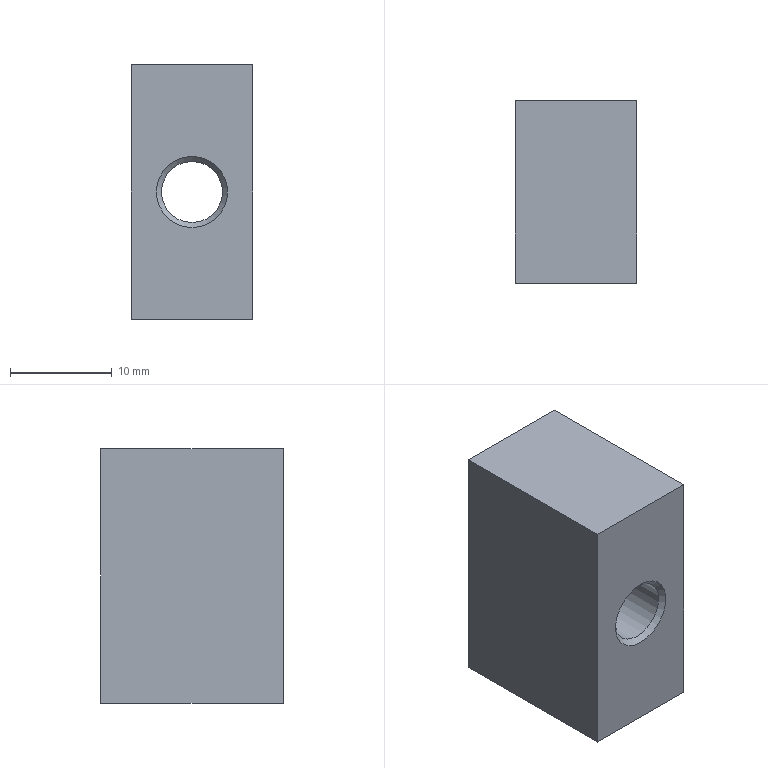Component | NX | SMALL_SLIDER | 1 solid | 9 faces | box 12 x 18 x 25 mm | volume 4886 mm3 | plane 6 | cone 2 | cylinder 1 | commonest cylinder face diameters 6 x1
STEP:
#1=CARTESIAN_POINT('',(0.,0.,0.));
#2=DIRECTION('',(0.,0.,1.));
#3=DIRECTION('',(1.,0.,0.));
#4=AXIS2_PLACEMENT_3D('',#1,#2,#3);
#5=CARTESIAN_POINT('',(-0.,-32.,1.));
#6=VERTEX_POINT('',#5);
#7=CARTESIAN_POINT('',(-0.,-32.,4.5));
#8=DIRECTION('',(0.,1.,0.));
#9=DIRECTION('',(0.,0.,-1.));
#10=AXIS2_PLACEMENT_3D('',#7,#8,#9);
#11=CIRCLE('',#10,3.5);
#12=CARTESIAN_POINT('',(6.,-32.,-8.));
#13=DIRECTION('',(0.,-1.,0.));
#14=DIRECTION('',(0.,0.,-1.));
#15=AXIS2_PLACEMENT_3D('',#12,#13,#14);
#16=PLANE('',#15);
#17=CARTESIAN_POINT('',(-9.,-6.));
#18=CARTESIAN_POINT('',(-9.,-12.062));
#19=CARTESIAN_POINT('',(-14.25,-9.031));
#20=CARTESIAN_POINT('',(-19.5,-6.));
#21=CARTESIAN_POINT('',(-14.25,-2.969));
#22=CARTESIAN_POINT('',(-9.,0.06218));
#23=CARTESIAN_POINT('',(-9.,-6.));
#24=(BOUNDED_CURVE()B_SPLINE_CURVE(2,(#17,#18,#19,#20,#21,#22,#23),.UNSPECIFIED.,.T.,.F.)B_SPLINE_CURVE_WITH_KNOTS((1,2,2,2,2,1),(-2.094,0.,2.094,4.189,6.283,8.378),.UNSPECIFIED.)CURVE()GEOMETRIC_REPRESENTATION_ITEM()RATIONAL_B_SPLINE_CURVE((1.,0.5,1.,0.5,1.,0.5,1.))REPRESENTATION_ITEM(''));
#25=(GEOMETRIC_REPRESENTATION_CONTEXT(2)PARAMETRIC_REPRESENTATION_CONTEXT()REPRESENTATION_CONTEXT('',''));
#26=DEFINITIONAL_REPRESENTATION('',(#24),#25);
#27=PCURVE('',#16,#26);
#28=CARTESIAN_POINT('',(-0.,-32.,4.5));
#29=DIRECTION('',(0.,-1.,0.));
#30=DIRECTION('',(0.,0.,-1.));
#31=AXIS2_PLACEMENT_3D('',#28,#29,#30);
#32=CONICAL_SURFACE('',#31,3.5,0.7854);
#33=CARTESIAN_POINT('',(6.283,0.));
#34=DIRECTION('',(-1.,0.));
#35=VECTOR('',#34,1.);
#36=LINE('',#33,#35);
#37=(GEOMETRIC_REPRESENTATION_CONTEXT(2)PARAMETRIC_REPRESENTATION_CONTEXT()REPRESENTATION_CONTEXT('',''));
#38=DEFINITIONAL_REPRESENTATION('',(#36),#37);
#39=PCURVE('',#32,#38);
#40=SURFACE_CURVE('',#11,(#27,#39),.PCURVE_S1.);
#41=EDGE_CURVE('',#6,#6,#40,.T.);
#42=ORIENTED_EDGE('',*,*,#41,.T.);
#43=EDGE_LOOP('',(#42));
#44=FACE_BOUND('',#43,.T.);
#45=CARTESIAN_POINT('',(-6.,-32.,-8.));
#46=VERTEX_POINT('',#45);
#47=CARTESIAN_POINT('',(-6.,-32.,17.));
#48=VERTEX_POINT('',#47);
#49=CARTESIAN_POINT('',(-6.,-32.,-8.));
#50=DIRECTION('',(0.,0.,1.));
#51=VECTOR('',#50,1.);
#52=LINE('',#49,#51);
#53=CARTESIAN_POINT('',(0.,-12.));
#54=DIRECTION('',(-1.,0.));
#55=VECTOR('',#54,1.);
#56=LINE('',#53,#55);
#57=(GEOMETRIC_REPRESENTATION_CONTEXT(2)PARAMETRIC_REPRESENTATION_CONTEXT()REPRESENTATION_CONTEXT('',''));
#58=DEFINITIONAL_REPRESENTATION('',(#56),#57);
#59=PCURVE('',#16,#58);
#60=CARTESIAN_POINT('',(-6.,-23.,4.5));
#61=DIRECTION('',(-1.,0.,0.));
#62=DIRECTION('',(0.,0.,1.));
#63=AXIS2_PLACEMENT_3D('',#60,#61,#62);
#64=PLANE('',#63);
#65=CARTESIAN_POINT('',(-12.5,-9.));
#66=DIRECTION('',(1.,0.));
#67=VECTOR('',#66,1.);
#68=LINE('',#65,#67);
#69=(GEOMETRIC_REPRESENTATION_CONTEXT(2)PARAMETRIC_REPRESENTATION_CONTEXT()REPRESENTATION_CONTEXT('',''));
#70=DEFINITIONAL_REPRESENTATION('',(#68),#69);
#71=PCURVE('',#64,#70);
#72=SURFACE_CURVE('',#52,(#59,#71),.PCURVE_S1.);
#73=EDGE_CURVE('',#46,#48,#72,.T.);
#74=ORIENTED_EDGE('',*,*,#73,.F.);
#75=CARTESIAN_POINT('',(6.,-32.,-8.));
#76=VERTEX_POINT('',#75);
#77=CARTESIAN_POINT('',(6.,-32.,-8.));
#78=DIRECTION('',(-1.,0.,0.));
#79=VECTOR('',#78,1.);
#80=LINE('',#77,#79);
#81=CARTESIAN_POINT('',(0.,0.));
#82=DIRECTION('',(0.,-1.));
#83=VECTOR('',#82,1.);
#84=LINE('',#81,#83);
#85=(GEOMETRIC_REPRESENTATION_CONTEXT(2)PARAMETRIC_REPRESENTATION_CONTEXT()REPRESENTATION_CONTEXT('',''));
#86=DEFINITIONAL_REPRESENTATION('',(#84),#85);
#87=PCURVE('',#16,#86);
#88=CARTESIAN_POINT('',(6.,-14.,-8.));
#89=DIRECTION('',(0.,0.,-1.));
#90=DIRECTION('',(-1.,0.,0.));
#91=AXIS2_PLACEMENT_3D('',#88,#89,#90);
#92=PLANE('',#91);
#93=CARTESIAN_POINT('',(0.,-18.));
#94=DIRECTION('',(1.,0.));
#95=VECTOR('',#94,1.);
#96=LINE('',#93,#95);
#97=(GEOMETRIC_REPRESENTATION_CONTEXT(2)PARAMETRIC_REPRESENTATION_CONTEXT()REPRESENTATION_CONTEXT('',''));
#98=DEFINITIONAL_REPRESENTATION('',(#96),#97);
#99=PCURVE('',#92,#98);
#100=SURFACE_CURVE('',#80,(#87,#99),.PCURVE_S1.);
#101=EDGE_CURVE('',#76,#46,#100,.T.);
#102=ORIENTED_EDGE('',*,*,#101,.F.);
#103=CARTESIAN_POINT('',(6.,-32.,17.));
#104=VERTEX_POINT('',#103);
#105=CARTESIAN_POINT('',(6.,-32.,-8.));
#106=DIRECTION('',(0.,0.,1.));
#107=VECTOR('',#106,1.);
#108=LINE('',#105,#107);
#109=CARTESIAN_POINT('',(0.,0.));
#110=DIRECTION('',(-1.,0.));
#111=VECTOR('',#110,1.);
#112=LINE('',#109,#111);
#113=(GEOMETRIC_REPRESENTATION_CONTEXT(2)PARAMETRIC_REPRESENTATION_CONTEXT()REPRESENTATION_CONTEXT('',''));
#114=DEFINITIONAL_REPRESENTATION('',(#112),#113);
#115=PCURVE('',#16,#114);
#116=CARTESIAN_POINT('',(6.,-23.,4.5));
#117=DIRECTION('',(-1.,0.,0.));
#118=DIRECTION('',(0.,0.,1.));
#119=AXIS2_PLACEMENT_3D('',#116,#117,#118);
#120=PLANE('',#119);
#121=CARTESIAN_POINT('',(-12.5,-9.));
#122=DIRECTION('',(1.,0.));
#123=VECTOR('',#122,1.);
#124=LINE('',#121,#123);
#125=(GEOMETRIC_REPRESENTATION_CONTEXT(2)PARAMETRIC_REPRESENTATION_CONTEXT()REPRESENTATION_CONTEXT('',''));
#126=DEFINITIONAL_REPRESENTATION('',(#124),#125);
#127=PCURVE('',#120,#126);
#128=SURFACE_CURVE('',#108,(#115,#127),.PCURVE_S1.);
#129=EDGE_CURVE('',#76,#104,#128,.T.);
#130=ORIENTED_EDGE('',*,*,#129,.T.);
#131=CARTESIAN_POINT('',(6.,-32.,17.));
#132=DIRECTION('',(-1.,0.,0.));
#133=VECTOR('',#132,1.);
#134=LINE('',#131,#133);
#135=CARTESIAN_POINT('',(-25.,0.));
#136=DIRECTION('',(0.,-1.));
#137=VECTOR('',#136,1.);
#138=LINE('',#135,#137);
#139=(GEOMETRIC_REPRESENTATION_CONTEXT(2)PARAMETRIC_REPRESENTATION_CONTEXT()REPRESENTATION_CONTEXT('',''));
#140=DEFINITIONAL_REPRESENTATION('',(#138),#139);
#141=PCURVE('',#16,#140);
#142=CARTESIAN_POINT('',(6.,-32.,17.));
#143=DIRECTION('',(0.,0.,1.));
#144=DIRECTION('',(1.,0.,0.));
#145=AXIS2_PLACEMENT_3D('',#142,#143,#144);
#146=PLANE('',#145);
#147=CARTESIAN_POINT('',(0.,0.));
#148=DIRECTION('',(-1.,0.));
#149=VECTOR('',#148,1.);
#150=LINE('',#147,#149);
#151=(GEOMETRIC_REPRESENTATION_CONTEXT(2)PARAMETRIC_REPRESENTATION_CONTEXT()REPRESENTATION_CONTEXT('',''));
#152=DEFINITIONAL_REPRESENTATION('',(#150),#151);
#153=PCURVE('',#146,#152);
#154=SURFACE_CURVE('',#134,(#141,#153),.PCURVE_S1.);
#155=EDGE_CURVE('',#104,#48,#154,.T.);
#156=ORIENTED_EDGE('',*,*,#155,.T.);
#157=EDGE_LOOP('',(#74,#102,#130,#156));
#158=FACE_BOUND('',#157,.T.);
#159=ADVANCED_FACE('',(#44,#158),#16,.T.);
#160=CARTESIAN_POINT('',(-6.,-14.,17.));
#161=VERTEX_POINT('',#160);
#162=CARTESIAN_POINT('',(-6.,-32.,17.));
#163=DIRECTION('',(0.,1.,0.));
#164=VECTOR('',#163,1.);
#165=LINE('',#162,#164);
#166=CARTESIAN_POINT('',(-12.,0.));
#167=DIRECTION('',(0.,1.));
#168=VECTOR('',#167,1.);
#169=LINE('',#166,#168);
#170=(GEOMETRIC_REPRESENTATION_CONTEXT(2)PARAMETRIC_REPRESENTATION_CONTEXT()REPRESENTATION_CONTEXT('',''));
#171=DEFINITIONAL_REPRESENTATION('',(#169),#170);
#172=PCURVE('',#146,#171);
#173=CARTESIAN_POINT('',(12.5,-9.));
#174=DIRECTION('',(0.,1.));
#175=VECTOR('',#174,1.);
#176=LINE('',#173,#175);
#177=(GEOMETRIC_REPRESENTATION_CONTEXT(2)PARAMETRIC_REPRESENTATION_CONTEXT()REPRESENTATION_CONTEXT('',''));
#178=DEFINITIONAL_REPRESENTATION('',(#176),#177);
#179=PCURVE('',#64,#178);
#180=SURFACE_CURVE('',#165,(#172,#179),.PCURVE_S1.);
#181=EDGE_CURVE('',#48,#161,#180,.T.);
#182=ORIENTED_EDGE('',*,*,#181,.F.);
#183=ORIENTED_EDGE('',*,*,#155,.F.);
#184=CARTESIAN_POINT('',(6.,-14.,17.));
#185=VERTEX_POINT('',#184);
#186=CARTESIAN_POINT('',(6.,-32.,17.));
#187=DIRECTION('',(0.,1.,0.));
#188=VECTOR('',#187,1.);
#189=LINE('',#186,#188);
#190=CARTESIAN_POINT('',(0.,0.));
#191=DIRECTION('',(0.,1.));
#192=VECTOR('',#191,1.);
#193=LINE('',#190,#192);
#194=(GEOMETRIC_REPRESENTATION_CONTEXT(2)PARAMETRIC_REPRESENTATION_CONTEXT()REPRESENTATION_CONTEXT('',''));
#195=DEFINITIONAL_REPRESENTATION('',(#193),#194);
#196=PCURVE('',#146,#195);
#197=CARTESIAN_POINT('',(12.5,-9.));
#198=DIRECTION('',(0.,1.));
#199=VECTOR('',#198,1.);
#200=LINE('',#197,#199);
#201=(GEOMETRIC_REPRESENTATION_CONTEXT(2)PARAMETRIC_REPRESENTATION_CONTEXT()REPRESENTATION_CONTEXT('',''));
#202=DEFINITIONAL_REPRESENTATION('',(#200),#201);
#203=PCURVE('',#120,#202);
#204=SURFACE_CURVE('',#189,(#196,#203),.PCURVE_S1.);
#205=EDGE_CURVE('',#104,#185,#204,.T.);
#206=ORIENTED_EDGE('',*,*,#205,.T.);
#207=CARTESIAN_POINT('',(6.,-14.,17.));
#208=DIRECTION('',(-1.,0.,0.));
#209=VECTOR('',#208,1.);
#210=LINE('',#207,#209);
#211=CARTESIAN_POINT('',(0.,18.));
#212=DIRECTION('',(-1.,0.));
#213=VECTOR('',#212,1.);
#214=LINE('',#211,#213);
#215=(GEOMETRIC_REPRESENTATION_CONTEXT(2)PARAMETRIC_REPRESENTATION_CONTEXT()REPRESENTATION_CONTEXT('',''));
#216=DEFINITIONAL_REPRESENTATION('',(#214),#215);
#217=PCURVE('',#146,#216);
#218=CARTESIAN_POINT('',(6.,-14.,17.));
#219=DIRECTION('',(0.,1.,0.));
#220=DIRECTION('',(0.,0.,1.));
#221=AXIS2_PLACEMENT_3D('',#218,#219,#220);
#222=PLANE('',#221);
#223=CARTESIAN_POINT('',(0.,0.));
#224=DIRECTION('',(0.,-1.));
#225=VECTOR('',#224,1.);
#226=LINE('',#223,#225);
#227=(GEOMETRIC_REPRESENTATION_CONTEXT(2)PARAMETRIC_REPRESENTATION_CONTEXT()REPRESENTATION_CONTEXT('',''));
#228=DEFINITIONAL_REPRESENTATION('',(#226),#227);
#229=PCURVE('',#222,#228);
#230=SURFACE_CURVE('',#210,(#217,#229),.PCURVE_S1.);
#231=EDGE_CURVE('',#185,#161,#230,.T.);
#232=ORIENTED_EDGE('',*,*,#231,.T.);
#233=EDGE_LOOP('',(#182,#183,#206,#232));
#234=FACE_BOUND('',#233,.T.);
#235=ADVANCED_FACE('',(#234),#146,.T.);
#236=CARTESIAN_POINT('',(-0.,-14.,8.));
#237=VERTEX_POINT('',#236);
#238=CARTESIAN_POINT('',(-0.,-14.,4.5));
#239=DIRECTION('',(0.,-1.,0.));
#240=DIRECTION('',(0.,0.,1.));
#241=AXIS2_PLACEMENT_3D('',#238,#239,#240);
#242=CIRCLE('',#241,3.5);
#243=CARTESIAN_POINT('',(-9.,-6.));
#244=CARTESIAN_POINT('',(-9.,-12.062));
#245=CARTESIAN_POINT('',(-14.25,-9.031));
#246=CARTESIAN_POINT('',(-19.5,-6.));
#247=CARTESIAN_POINT('',(-14.25,-2.969));
#248=CARTESIAN_POINT('',(-9.,0.06218));
#249=CARTESIAN_POINT('',(-9.,-6.));
#250=(BOUNDED_CURVE()B_SPLINE_CURVE(2,(#243,#244,#245,#246,#247,#248,#249),.UNSPECIFIED.,.T.,.F.)B_SPLINE_CURVE_WITH_KNOTS((1,2,2,2,2,1),(-2.094,0.,2.094,4.189,6.283,8.378),.UNSPECIFIED.)CURVE()GEOMETRIC_REPRESENTATION_ITEM()RATIONAL_B_SPLINE_CURVE((1.,0.5,1.,0.5,1.,0.5,1.))REPRESENTATION_ITEM(''));
#251=(GEOMETRIC_REPRESENTATION_CONTEXT(2)PARAMETRIC_REPRESENTATION_CONTEXT()REPRESENTATION_CONTEXT('',''));
#252=DEFINITIONAL_REPRESENTATION('',(#250),#251);
#253=PCURVE('',#222,#252);
#254=CARTESIAN_POINT('',(-0.,-14.,4.5));
#255=DIRECTION('',(0.,1.,0.));
#256=DIRECTION('',(0.,0.,1.));
#257=AXIS2_PLACEMENT_3D('',#254,#255,#256);
#258=CONICAL_SURFACE('',#257,3.5,0.7854);
#259=CARTESIAN_POINT('',(6.283,0.));
#260=DIRECTION('',(-1.,0.));
#261=VECTOR('',#260,1.);
#262=LINE('',#259,#261);
#263=(GEOMETRIC_REPRESENTATION_CONTEXT(2)PARAMETRIC_REPRESENTATION_CONTEXT()REPRESENTATION_CONTEXT('',''));
#264=DEFINITIONAL_REPRESENTATION('',(#262),#263);
#265=PCURVE('',#258,#264);
#266=SURFACE_CURVE('',#242,(#253,#265),.PCURVE_S1.);
#267=EDGE_CURVE('',#237,#237,#266,.T.);
#268=ORIENTED_EDGE('',*,*,#267,.T.);
#269=EDGE_LOOP('',(#268));
#270=FACE_BOUND('',#269,.T.);
#271=CARTESIAN_POINT('',(-6.,-14.,-8.));
#272=VERTEX_POINT('',#271);
#273=CARTESIAN_POINT('',(-6.,-14.,17.));
#274=DIRECTION('',(0.,0.,-1.));
#275=VECTOR('',#274,1.);
#276=LINE('',#273,#275);
#277=CARTESIAN_POINT('',(0.,-12.));
#278=DIRECTION('',(-1.,0.));
#279=VECTOR('',#278,1.);
#280=LINE('',#277,#279);
#281=(GEOMETRIC_REPRESENTATION_CONTEXT(2)PARAMETRIC_REPRESENTATION_CONTEXT()REPRESENTATION_CONTEXT('',''));
#282=DEFINITIONAL_REPRESENTATION('',(#280),#281);
#283=PCURVE('',#222,#282);
#284=CARTESIAN_POINT('',(12.5,9.));
#285=DIRECTION('',(-1.,0.));
#286=VECTOR('',#285,1.);
#287=LINE('',#284,#286);
#288=(GEOMETRIC_REPRESENTATION_CONTEXT(2)PARAMETRIC_REPRESENTATION_CONTEXT()REPRESENTATION_CONTEXT('',''));
#289=DEFINITIONAL_REPRESENTATION('',(#287),#288);
#290=PCURVE('',#64,#289);
#291=SURFACE_CURVE('',#276,(#283,#290),.PCURVE_S1.);
#292=EDGE_CURVE('',#161,#272,#291,.T.);
#293=ORIENTED_EDGE('',*,*,#292,.F.);
#294=ORIENTED_EDGE('',*,*,#231,.F.);
#295=CARTESIAN_POINT('',(6.,-14.,-8.));
#296=VERTEX_POINT('',#295);
#297=CARTESIAN_POINT('',(6.,-14.,17.));
#298=DIRECTION('',(0.,0.,-1.));
#299=VECTOR('',#298,1.);
#300=LINE('',#297,#299);
#301=CARTESIAN_POINT('',(0.,0.));
#302=DIRECTION('',(-1.,0.));
#303=VECTOR('',#302,1.);
#304=LINE('',#301,#303);
#305=(GEOMETRIC_REPRESENTATION_CONTEXT(2)PARAMETRIC_REPRESENTATION_CONTEXT()REPRESENTATION_CONTEXT('',''));
#306=DEFINITIONAL_REPRESENTATION('',(#304),#305);
#307=PCURVE('',#222,#306);
#308=CARTESIAN_POINT('',(12.5,9.));
#309=DIRECTION('',(-1.,0.));
#310=VECTOR('',#309,1.);
#311=LINE('',#308,#310);
#312=(GEOMETRIC_REPRESENTATION_CONTEXT(2)PARAMETRIC_REPRESENTATION_CONTEXT()REPRESENTATION_CONTEXT('',''));
#313=DEFINITIONAL_REPRESENTATION('',(#311),#312);
#314=PCURVE('',#120,#313);
#315=SURFACE_CURVE('',#300,(#307,#314),.PCURVE_S1.);
#316=EDGE_CURVE('',#185,#296,#315,.T.);
#317=ORIENTED_EDGE('',*,*,#316,.T.);
#318=CARTESIAN_POINT('',(6.,-14.,-8.));
#319=DIRECTION('',(-1.,0.,0.));
#320=VECTOR('',#319,1.);
#321=LINE('',#318,#320);
#322=CARTESIAN_POINT('',(-25.,0.));
#323=DIRECTION('',(0.,-1.));
#324=VECTOR('',#323,1.);
#325=LINE('',#322,#324);
#326=(GEOMETRIC_REPRESENTATION_CONTEXT(2)PARAMETRIC_REPRESENTATION_CONTEXT()REPRESENTATION_CONTEXT('',''));
#327=DEFINITIONAL_REPRESENTATION('',(#325),#326);
#328=PCURVE('',#222,#327);
#329=CARTESIAN_POINT('',(0.,0.));
#330=DIRECTION('',(1.,0.));
#331=VECTOR('',#330,1.);
#332=LINE('',#329,#331);
#333=(GEOMETRIC_REPRESENTATION_CONTEXT(2)PARAMETRIC_REPRESENTATION_CONTEXT()REPRESENTATION_CONTEXT('',''));
#334=DEFINITIONAL_REPRESENTATION('',(#332),#333);
#335=PCURVE('',#92,#334);
#336=SURFACE_CURVE('',#321,(#328,#335),.PCURVE_S1.);
#337=EDGE_CURVE('',#296,#272,#336,.T.);
#338=ORIENTED_EDGE('',*,*,#337,.T.);
#339=EDGE_LOOP('',(#293,#294,#317,#338));
#340=FACE_BOUND('',#339,.T.);
#341=ADVANCED_FACE('',(#270,#340),#222,.T.);
#342=CARTESIAN_POINT('',(-6.,-14.,-8.));
#343=DIRECTION('',(0.,-1.,0.));
#344=VECTOR('',#343,1.);
#345=LINE('',#342,#344);
#346=CARTESIAN_POINT('',(12.,0.));
#347=DIRECTION('',(0.,-1.));
#348=VECTOR('',#347,1.);
#349=LINE('',#346,#348);
#350=(GEOMETRIC_REPRESENTATION_CONTEXT(2)PARAMETRIC_REPRESENTATION_CONTEXT()REPRESENTATION_CONTEXT('',''));
#351=DEFINITIONAL_REPRESENTATION('',(#349),#350);
#352=PCURVE('',#92,#351);
#353=CARTESIAN_POINT('',(-12.5,9.));
#354=DIRECTION('',(0.,-1.));
#355=VECTOR('',#354,1.);
#356=LINE('',#353,#355);
#357=(GEOMETRIC_REPRESENTATION_CONTEXT(2)PARAMETRIC_REPRESENTATION_CONTEXT()REPRESENTATION_CONTEXT('',''));
#358=DEFINITIONAL_REPRESENTATION('',(#356),#357);
#359=PCURVE('',#64,#358);
#360=SURFACE_CURVE('',#345,(#352,#359),.PCURVE_S1.);
#361=EDGE_CURVE('',#272,#46,#360,.T.);
#362=ORIENTED_EDGE('',*,*,#361,.F.);
#363=ORIENTED_EDGE('',*,*,#337,.F.);
#364=CARTESIAN_POINT('',(6.,-14.,-8.));
#365=DIRECTION('',(0.,-1.,0.));
#366=VECTOR('',#365,1.);
#367=LINE('',#364,#366);
#368=CARTESIAN_POINT('',(0.,0.));
#369=DIRECTION('',(0.,-1.));
#370=VECTOR('',#369,1.);
#371=LINE('',#368,#370);
#372=(GEOMETRIC_REPRESENTATION_CONTEXT(2)PARAMETRIC_REPRESENTATION_CONTEXT()REPRESENTATION_CONTEXT('',''));
#373=DEFINITIONAL_REPRESENTATION('',(#371),#372);
#374=PCURVE('',#92,#373);
#375=CARTESIAN_POINT('',(-12.5,9.));
#376=DIRECTION('',(0.,-1.));
#377=VECTOR('',#376,1.);
#378=LINE('',#375,#377);
#379=(GEOMETRIC_REPRESENTATION_CONTEXT(2)PARAMETRIC_REPRESENTATION_CONTEXT()REPRESENTATION_CONTEXT('',''));
#380=DEFINITIONAL_REPRESENTATION('',(#378),#379);
#381=PCURVE('',#120,#380);
#382=SURFACE_CURVE('',#367,(#374,#381),.PCURVE_S1.);
#383=EDGE_CURVE('',#296,#76,#382,.T.);
#384=ORIENTED_EDGE('',*,*,#383,.T.);
#385=ORIENTED_EDGE('',*,*,#101,.T.);
#386=EDGE_LOOP('',(#362,#363,#384,#385));
#387=FACE_BOUND('',#386,.T.);
#388=ADVANCED_FACE('',(#387),#92,.T.);
#389=ORIENTED_EDGE('',*,*,#129,.F.);
#390=ORIENTED_EDGE('',*,*,#383,.F.);
#391=ORIENTED_EDGE('',*,*,#316,.F.);
#392=ORIENTED_EDGE('',*,*,#205,.F.);
#393=EDGE_LOOP('',(#389,#390,#391,#392));
#394=FACE_BOUND('',#393,.T.);
#395=ADVANCED_FACE('',(#394),#120,.F.);
#396=ORIENTED_EDGE('',*,*,#73,.T.);
#397=ORIENTED_EDGE('',*,*,#181,.T.);
#398=ORIENTED_EDGE('',*,*,#292,.T.);
#399=ORIENTED_EDGE('',*,*,#361,.T.);
#400=EDGE_LOOP('',(#396,#397,#398,#399));
#401=FACE_BOUND('',#400,.T.);
#402=ADVANCED_FACE('',(#401),#64,.T.);
#403=CARTESIAN_POINT('',(-0.,-14.5,7.5));
#404=VERTEX_POINT('',#403);
#405=CARTESIAN_POINT('',(-0.,-14.5,4.5));
#406=DIRECTION('',(0.,1.,0.));
#407=DIRECTION('',(0.,0.,1.));
#408=AXIS2_PLACEMENT_3D('',#405,#406,#407);
#409=CIRCLE('',#408,3.);
#410=CARTESIAN_POINT('',(-0.,-43.,4.5));
#411=DIRECTION('',(0.,1.,0.));
#412=DIRECTION('',(0.,0.,1.));
#413=AXIS2_PLACEMENT_3D('',#410,#411,#412);
#414=CYLINDRICAL_SURFACE('',#413,3.);
#415=CARTESIAN_POINT('',(0.,28.5));
#416=DIRECTION('',(1.,0.));
#417=VECTOR('',#416,1.);
#418=LINE('',#415,#417);
#419=(GEOMETRIC_REPRESENTATION_CONTEXT(2)PARAMETRIC_REPRESENTATION_CONTEXT()REPRESENTATION_CONTEXT('',''));
#420=DEFINITIONAL_REPRESENTATION('',(#418),#419);
#421=PCURVE('',#414,#420);
#422=CARTESIAN_POINT('',(0.,-0.5));
#423=DIRECTION('',(1.,0.));
#424=VECTOR('',#423,1.);
#425=LINE('',#422,#424);
#426=(GEOMETRIC_REPRESENTATION_CONTEXT(2)PARAMETRIC_REPRESENTATION_CONTEXT()REPRESENTATION_CONTEXT('',''));
#427=DEFINITIONAL_REPRESENTATION('',(#425),#426);
#428=PCURVE('',#258,#427);
#429=SURFACE_CURVE('',#409,(#421,#428),.PCURVE_S1.);
#430=EDGE_CURVE('',#404,#404,#429,.T.);
#431=ORIENTED_EDGE('',*,*,#430,.F.);
#432=CARTESIAN_POINT('',(-0.,-31.5,7.5));
#433=VERTEX_POINT('',#432);
#434=CARTESIAN_POINT('',(-0.,-31.5,7.5));
#435=CARTESIAN_POINT('',(-0.,-14.5,7.5));
#436=B_SPLINE_CURVE_WITH_KNOTS('',1,(#434,#435),.UNSPECIFIED.,.F.,.F.,(2,2),(11.5,28.5),.PIECEWISE_BEZIER_KNOTS.);
#437=CARTESIAN_POINT('',(0.,0.));
#438=DIRECTION('',(0.,1.));
#439=VECTOR('',#438,1.);
#440=LINE('',#437,#439);
#441=(GEOMETRIC_REPRESENTATION_CONTEXT(2)PARAMETRIC_REPRESENTATION_CONTEXT()REPRESENTATION_CONTEXT('',''));
#442=DEFINITIONAL_REPRESENTATION('',(#440),#441);
#443=PCURVE('',#414,#442);
#444=CARTESIAN_POINT('',(6.283,0.));
#445=DIRECTION('',(0.,1.));
#446=VECTOR('',#445,1.);
#447=LINE('',#444,#446);
#448=(GEOMETRIC_REPRESENTATION_CONTEXT(2)PARAMETRIC_REPRESENTATION_CONTEXT()REPRESENTATION_CONTEXT('',''));
#449=DEFINITIONAL_REPRESENTATION('',(#447),#448);
#450=PCURVE('',#414,#449);
#451=SEAM_CURVE('',#436,(#443,#450),.PCURVE_S1.);
#452=EDGE_CURVE('',#433,#404,#451,.T.);
#453=ORIENTED_EDGE('',*,*,#452,.F.);
#454=CARTESIAN_POINT('',(-0.,-31.5,1.5));
#455=VERTEX_POINT('',#454);
#456=CARTESIAN_POINT('',(-0.,-31.5,4.5));
#457=DIRECTION('',(0.,-1.,0.));
#458=DIRECTION('',(0.,0.,-1.));
#459=AXIS2_PLACEMENT_3D('',#456,#457,#458);
#460=CIRCLE('',#459,3.);
#461=CARTESIAN_POINT('',(3.142,11.5));
#462=DIRECTION('',(-1.,0.));
#463=VECTOR('',#462,1.);
#464=LINE('',#461,#463);
#465=(GEOMETRIC_REPRESENTATION_CONTEXT(2)PARAMETRIC_REPRESENTATION_CONTEXT()REPRESENTATION_CONTEXT('',''));
#466=DEFINITIONAL_REPRESENTATION('',(#464),#465);
#467=PCURVE('',#414,#466);
#468=CARTESIAN_POINT('',(0.,-0.5));
#469=DIRECTION('',(1.,0.));
#470=VECTOR('',#469,1.);
#471=LINE('',#468,#470);
#472=(GEOMETRIC_REPRESENTATION_CONTEXT(2)PARAMETRIC_REPRESENTATION_CONTEXT()REPRESENTATION_CONTEXT('',''));
#473=DEFINITIONAL_REPRESENTATION('',(#471),#472);
#474=PCURVE('',#32,#473);
#475=SURFACE_CURVE('',#460,(#467,#474),.PCURVE_S1.);
#476=EDGE_CURVE('',#455,#433,#475,.T.);
#477=ORIENTED_EDGE('',*,*,#476,.F.);
#478=CARTESIAN_POINT('',(-0.,-31.5,4.5));
#479=DIRECTION('',(0.,-1.,0.));
#480=DIRECTION('',(0.,0.,-1.));
#481=AXIS2_PLACEMENT_3D('',#478,#479,#480);
#482=CIRCLE('',#481,3.);
#483=CARTESIAN_POINT('',(9.425,11.5));
#484=DIRECTION('',(-1.,0.));
#485=VECTOR('',#484,1.);
#486=LINE('',#483,#485);
#487=(GEOMETRIC_REPRESENTATION_CONTEXT(2)PARAMETRIC_REPRESENTATION_CONTEXT()REPRESENTATION_CONTEXT('',''));
#488=DEFINITIONAL_REPRESENTATION('',(#486),#487);
#489=PCURVE('',#414,#488);
#490=CARTESIAN_POINT('',(0.,-0.5));
#491=DIRECTION('',(1.,-0.));
#492=VECTOR('',#491,1.);
#493=LINE('',#490,#492);
#494=(GEOMETRIC_REPRESENTATION_CONTEXT(2)PARAMETRIC_REPRESENTATION_CONTEXT()REPRESENTATION_CONTEXT('',''));
#495=DEFINITIONAL_REPRESENTATION('',(#493),#494);
#496=PCURVE('',#32,#495);
#497=SURFACE_CURVE('',#482,(#489,#496),.PCURVE_S1.);
#498=EDGE_CURVE('',#433,#455,#497,.T.);
#499=ORIENTED_EDGE('',*,*,#498,.F.);
#500=ORIENTED_EDGE('',*,*,#452,.T.);
#501=EDGE_LOOP('',(#431,#453,#477,#499,#500));
#502=FACE_BOUND('',#501,.F.);
#503=ADVANCED_FACE('',(#502),#414,.F.);
#504=ORIENTED_EDGE('',*,*,#430,.T.);
#505=CARTESIAN_POINT('',(-0.,-14.5,7.5));
#506=CARTESIAN_POINT('',(-0.,-14.,8.));
#507=B_SPLINE_CURVE_WITH_KNOTS('',1,(#505,#506),.UNSPECIFIED.,.F.,.F.,(2,2),(-0.7071,0.),.PIECEWISE_BEZIER_KNOTS.);
#508=CARTESIAN_POINT('',(6.283,0.));
#509=DIRECTION('',(0.,1.));
#510=VECTOR('',#509,1.);
#511=LINE('',#508,#510);
#512=(GEOMETRIC_REPRESENTATION_CONTEXT(2)PARAMETRIC_REPRESENTATION_CONTEXT()REPRESENTATION_CONTEXT('',''));
#513=DEFINITIONAL_REPRESENTATION('',(#511),#512);
#514=PCURVE('',#258,#513);
#515=CARTESIAN_POINT('',(0.,0.));
#516=DIRECTION('',(0.,1.));
#517=VECTOR('',#516,1.);
#518=LINE('',#515,#517);
#519=(GEOMETRIC_REPRESENTATION_CONTEXT(2)PARAMETRIC_REPRESENTATION_CONTEXT()REPRESENTATION_CONTEXT('',''));
#520=DEFINITIONAL_REPRESENTATION('',(#518),#519);
#521=PCURVE('',#258,#520);
#522=SEAM_CURVE('',#507,(#514,#521),.PCURVE_S1.);
#523=EDGE_CURVE('',#404,#237,#522,.T.);
#524=ORIENTED_EDGE('',*,*,#523,.T.);
#525=ORIENTED_EDGE('',*,*,#267,.T.);
#526=ORIENTED_EDGE('',*,*,#523,.F.);
#527=EDGE_LOOP('',(#504,#524,#525,#526));
#528=FACE_BOUND('',#527,.F.);
#529=ADVANCED_FACE('',(#528),#258,.F.);
#530=ORIENTED_EDGE('',*,*,#498,.T.);
#531=CARTESIAN_POINT('',(-0.,-31.5,1.5));
#532=CARTESIAN_POINT('',(-0.,-32.,1.));
#533=B_SPLINE_CURVE_WITH_KNOTS('',1,(#531,#532),.UNSPECIFIED.,.F.,.F.,(2,2),(-0.7071,0.),.PIECEWISE_BEZIER_KNOTS.);
#534=CARTESIAN_POINT('',(6.283,0.));
#535=DIRECTION('',(0.,1.));
#536=VECTOR('',#535,1.);
#537=LINE('',#534,#536);
#538=(GEOMETRIC_REPRESENTATION_CONTEXT(2)PARAMETRIC_REPRESENTATION_CONTEXT()REPRESENTATION_CONTEXT('',''));
#539=DEFINITIONAL_REPRESENTATION('',(#537),#538);
#540=PCURVE('',#32,#539);
#541=CARTESIAN_POINT('',(0.,0.));
#542=DIRECTION('',(0.,1.));
#543=VECTOR('',#542,1.);
#544=LINE('',#541,#543);
#545=(GEOMETRIC_REPRESENTATION_CONTEXT(2)PARAMETRIC_REPRESENTATION_CONTEXT()REPRESENTATION_CONTEXT('',''));
#546=DEFINITIONAL_REPRESENTATION('',(#544),#545);
#547=PCURVE('',#32,#546);
#548=SEAM_CURVE('',#533,(#540,#547),.PCURVE_S1.);
#549=EDGE_CURVE('',#455,#6,#548,.T.);
#550=ORIENTED_EDGE('',*,*,#549,.T.);
#551=ORIENTED_EDGE('',*,*,#41,.T.);
#552=ORIENTED_EDGE('',*,*,#549,.F.);
#553=ORIENTED_EDGE('',*,*,#476,.T.);
#554=EDGE_LOOP('',(#530,#550,#551,#552,#553));
#555=FACE_BOUND('',#554,.F.);
#556=ADVANCED_FACE('',(#555),#32,.F.);
#557=CLOSED_SHELL('',(#159,#235,#341,#388,#395,#402,#503,#529,#556));
#558=MANIFOLD_SOLID_BREP('',#557);
#559=(LENGTH_UNIT()NAMED_UNIT(*)SI_UNIT(.MILLI.,.METRE.));
#560=UNCERTAINTY_MEASURE_WITH_UNIT(LENGTH_MEASURE(0.000002),#559,'','');
#561=(NAMED_UNIT(*)PLANE_ANGLE_UNIT()SI_UNIT($,.RADIAN.));
#562=(NAMED_UNIT(*)SI_UNIT($,.STERADIAN.)SOLID_ANGLE_UNIT());
#563=(GEOMETRIC_REPRESENTATION_CONTEXT(3)GLOBAL_UNCERTAINTY_ASSIGNED_CONTEXT((#560))GLOBAL_UNIT_ASSIGNED_CONTEXT((#559,#561,#562))REPRESENTATION_CONTEXT('',''));
#564=ADVANCED_BREP_SHAPE_REPRESENTATION('',(#4,#558),#563);